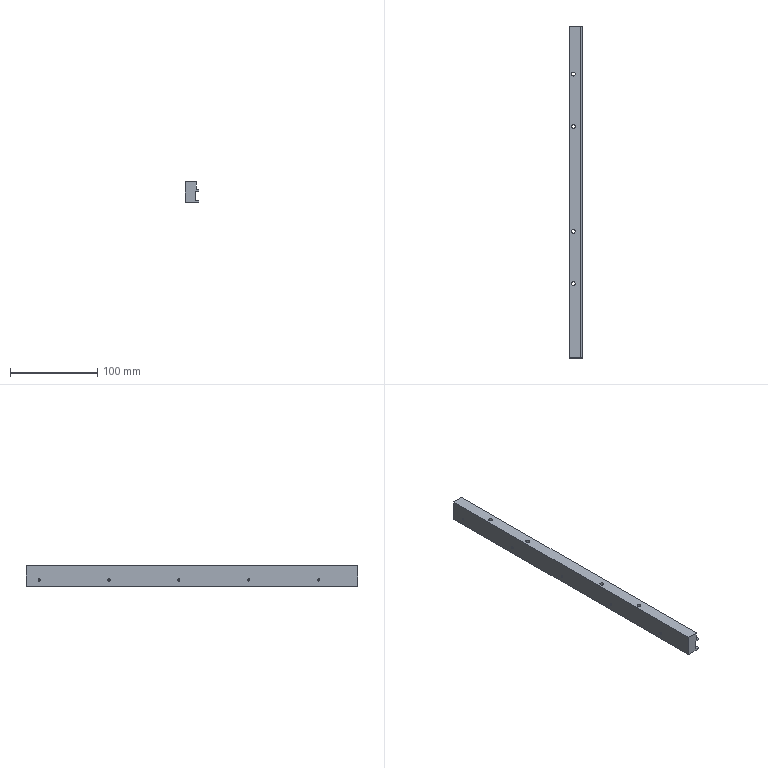Component | SolidWorks | AUTO-SpinDryWashing-01-03000008-3 | 1 solid | 56 faces | box 16 x 380 x 24 mm | volume 116570 mm3 | cylinder 28 | plane 16 | cone 12 | commonest cylinder face diameters 2.5 x12 8 x8 4.5 x8 | material AISI 304
build123d program:
from build123d import *

# Parameters (mm, degrees)
BOSS_EXTRUDE1_DEPTH                                  = 175
M3_TAPPED_HOLE1_D                                    = 2.5
M3_TAPPED_HOLE1_DEPTH                                = 7.5
M3_TAPPED_HOLE1_TIP                                  = 0.7511
SKETCH6_W                                            = 13
SKETCH6_H                                            = 350
BOSS_EXTRUDE2_DEPTH                                  = 9
HOLE_SIZE_ACCORDING_TO_HEX_SOCKET_HEAD_C_D           = 4.5
HOLE_SIZE_ACCORDING_TO_HEX_SOCKET_HEAD_C_CBORE_D     = 8
HOLE_SIZE_ACCORDING_TO_HEX_SOCKET_HEAD_C_CBORE_DEPTH = 10
BOSS_EXTRUDE3_DEPTH                                  = 30
M3_TAPPED_HOLE2_D                                    = 2.5
M3_TAPPED_HOLE2_DEPTH                                = 7.5
M3_TAPPED_HOLE2_TIP                                  = 0.7511


with BuildPart() as part:
    # Sketch1 → Boss-Extrude1 (new, symmetric)
    with BuildSketch(Plane.XY):
        Polygon((-8, -5.25), (-8, -7.5), (8, -7.5), (8, 7.5), (-8, 7.5), (-8, 5.25), (-4, 5.25), (-4, -5.25), align=None)
    extrude(amount=BOSS_EXTRUDE1_DEPTH, both=True)

    # M3 Tapped Hole1
    with Locations(Plane(origin=(8, 0, 0), x_dir=(0, 0, -1), z_dir=(1, 0, 0))):
        with Locations((160, 0), (80, 0), (0, 0), (-80, 0), (-160, 0)):
            Hole(M3_TAPPED_HOLE1_D / 2, depth=M3_TAPPED_HOLE1_DEPTH)
            with Locations((0, 0, -(M3_TAPPED_HOLE1_DEPTH + M3_TAPPED_HOLE1_TIP / 2))):  # 118° drill point
                Cone(0, M3_TAPPED_HOLE1_D / 2, M3_TAPPED_HOLE1_TIP, mode=Mode.SUBTRACT)

    # Sketch6 → Boss-Extrude2 (add)
    with BuildSketch(Plane.XZ.offset(7.5)):
        with Locations((1.5, 0)):
            Rectangle(SKETCH6_W, SKETCH6_H)
    extrude(amount=BOSS_EXTRUDE2_DEPTH)

    # Hole Size according to Hex Socket Head C (through all)
    with Locations(Plane(origin=(0, 7.5, 0), x_dir=(1, 0, 0), z_dir=(0, 1, 0))):
        with Locations((3, -120), (3, -60), (3, 60), (3, 120)):
            CounterBoreHole(HOLE_SIZE_ACCORDING_TO_HEX_SOCKET_HEAD_C_D / 2, HOLE_SIZE_ACCORDING_TO_HEX_SOCKET_HEAD_C_CBORE_D / 2, HOLE_SIZE_ACCORDING_TO_HEX_SOCKET_HEAD_C_CBORE_DEPTH)

    # Sketch7 → Boss-Extrude3 (add)
    with BuildSketch(Plane.XY.offset(175)):
        Polygon((-8, 5.25), (-4, 5.25), (-4, -5.25), (-8, -5.25), (-8, -7.5), (-5, -7.5), (-5, -16.5), (8, -16.5), (8, 7.5), (-8, 7.5), align=None)
    extrude(amount=BOSS_EXTRUDE3_DEPTH)

    # M3 Tapped Hole2
    with Locations(Plane.ZY.offset(4)):
        with Locations((195, -0.25)):
            Hole(M3_TAPPED_HOLE2_D / 2, depth=M3_TAPPED_HOLE2_DEPTH)
            with Locations((0, 0, -(M3_TAPPED_HOLE2_DEPTH + M3_TAPPED_HOLE2_TIP / 2))):  # 118° drill point
                Cone(0, M3_TAPPED_HOLE2_D / 2, M3_TAPPED_HOLE2_TIP, mode=Mode.SUBTRACT)


solid = part.part

# Placed as in the assembly
solid = solid.moved(Location((-357, 643, 57.5), (90, 0, -180)))